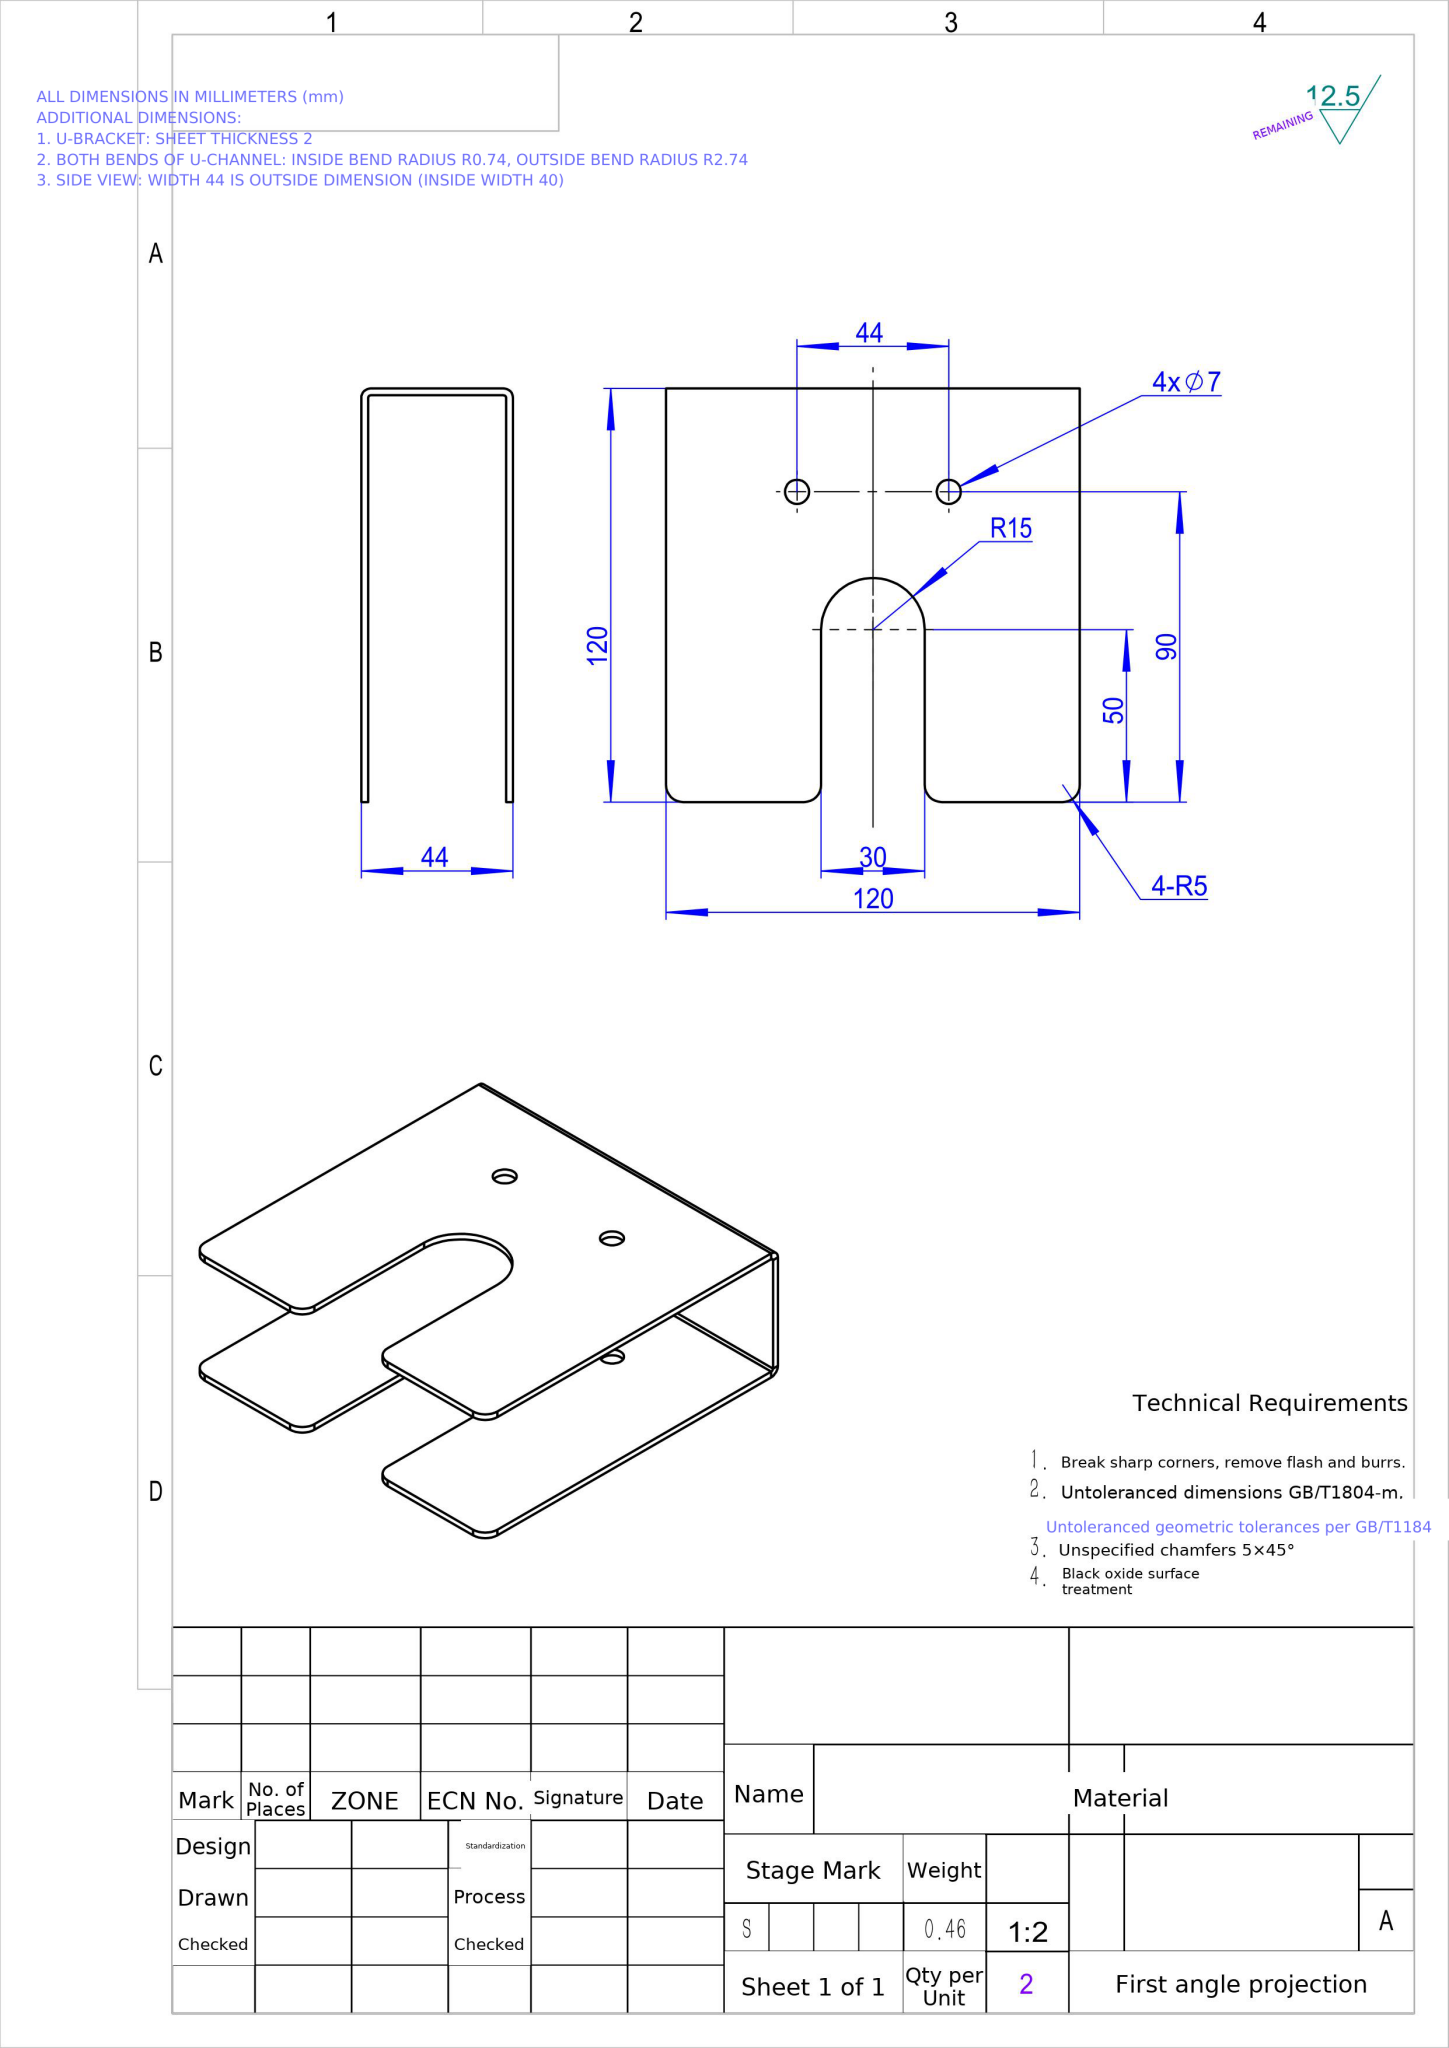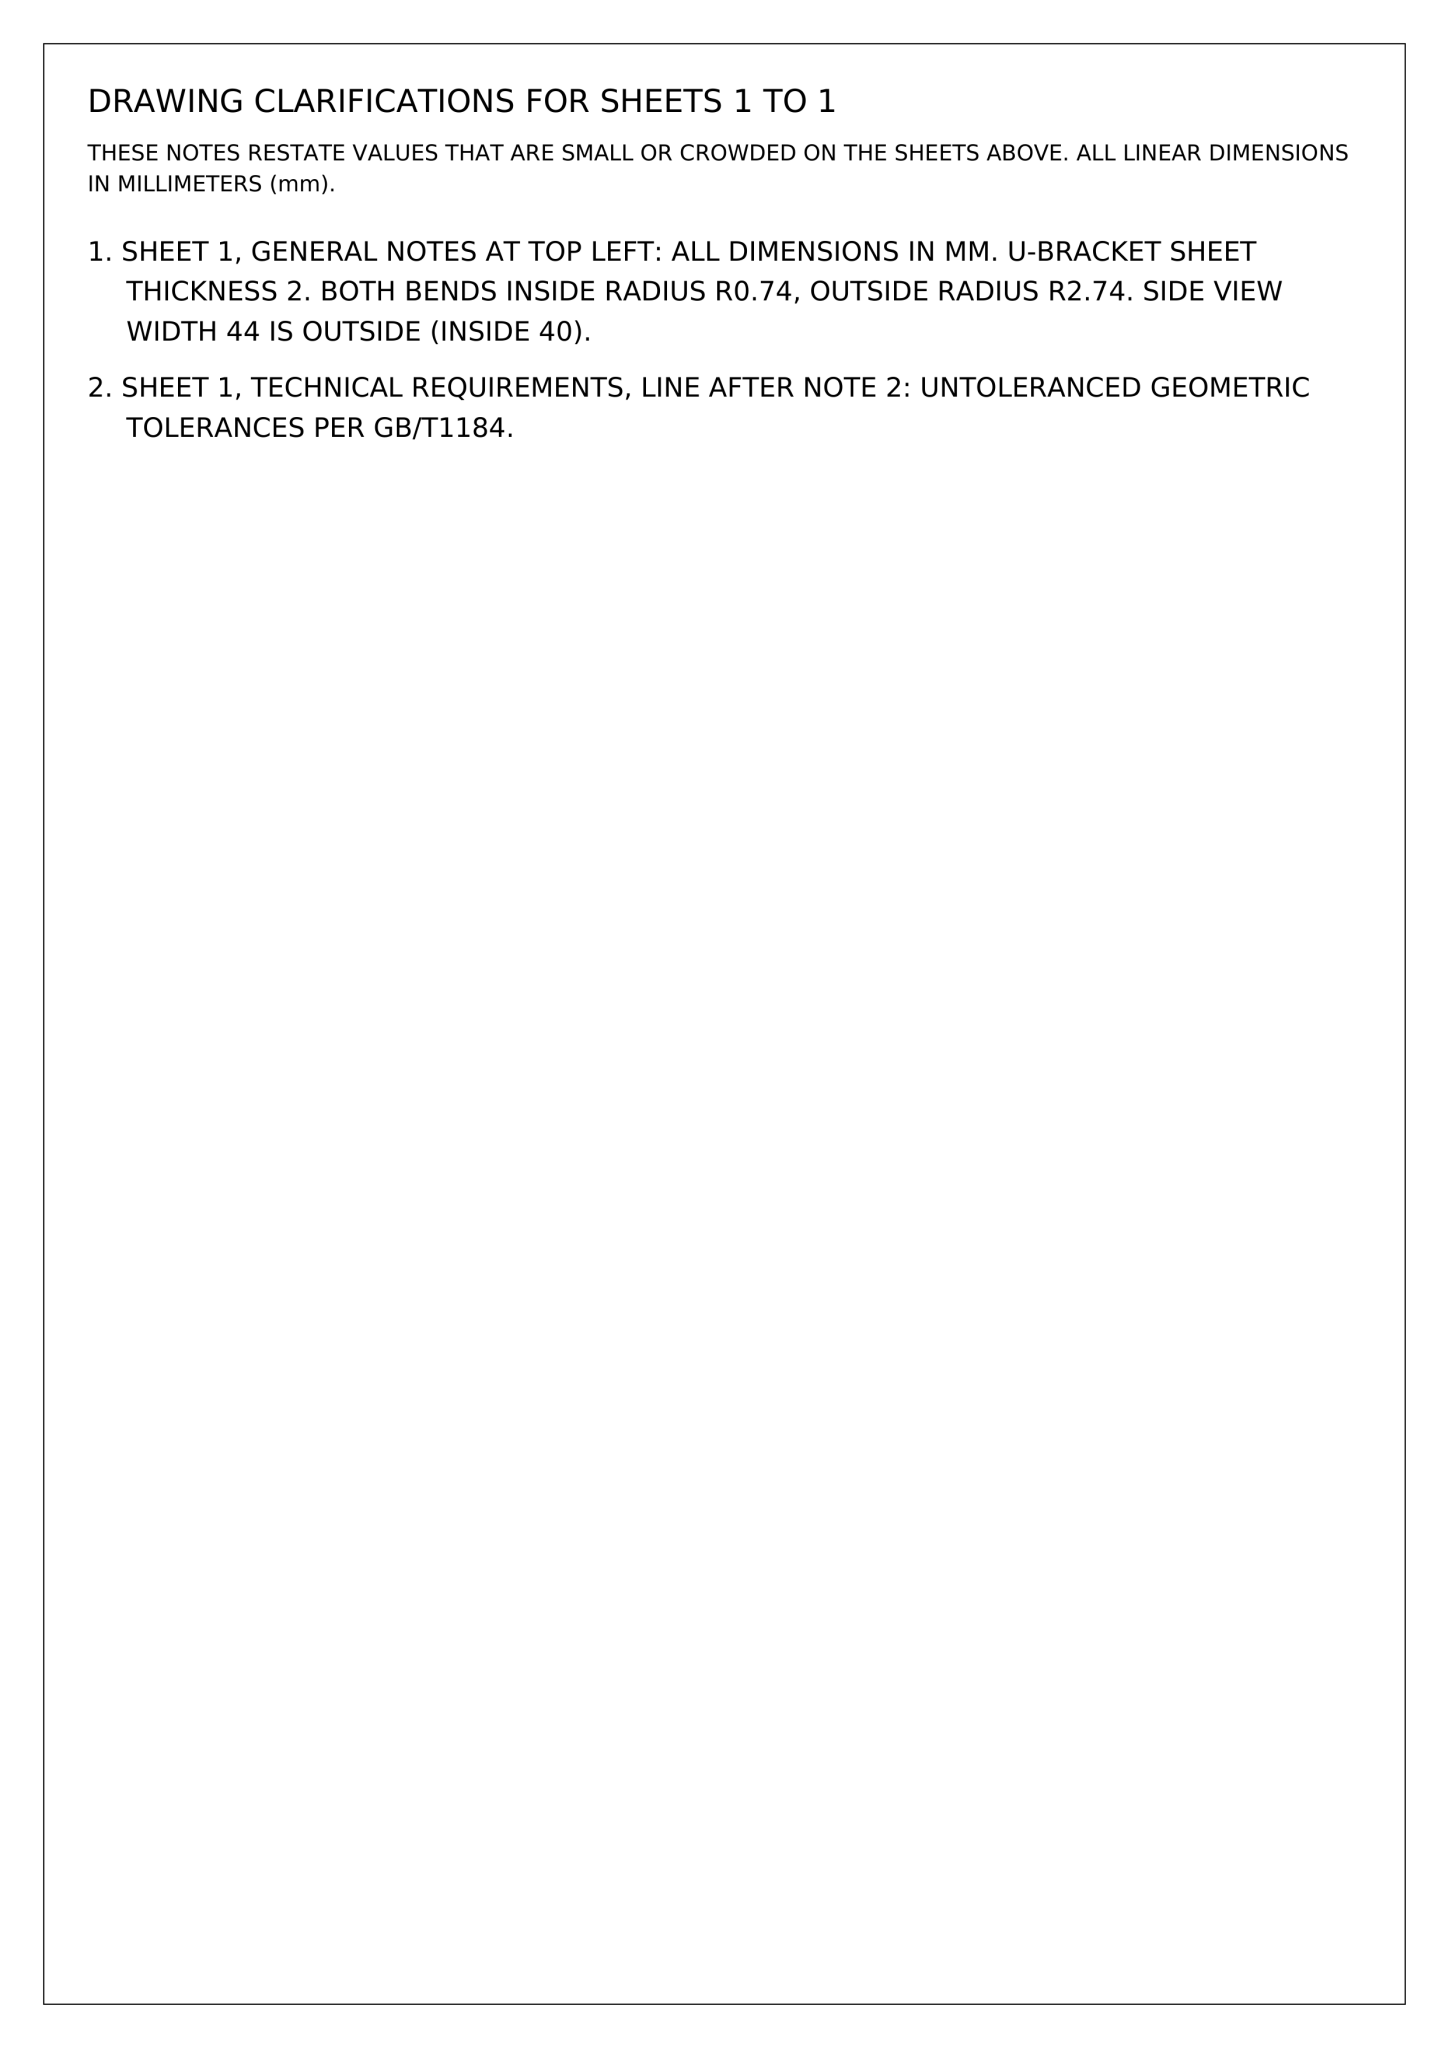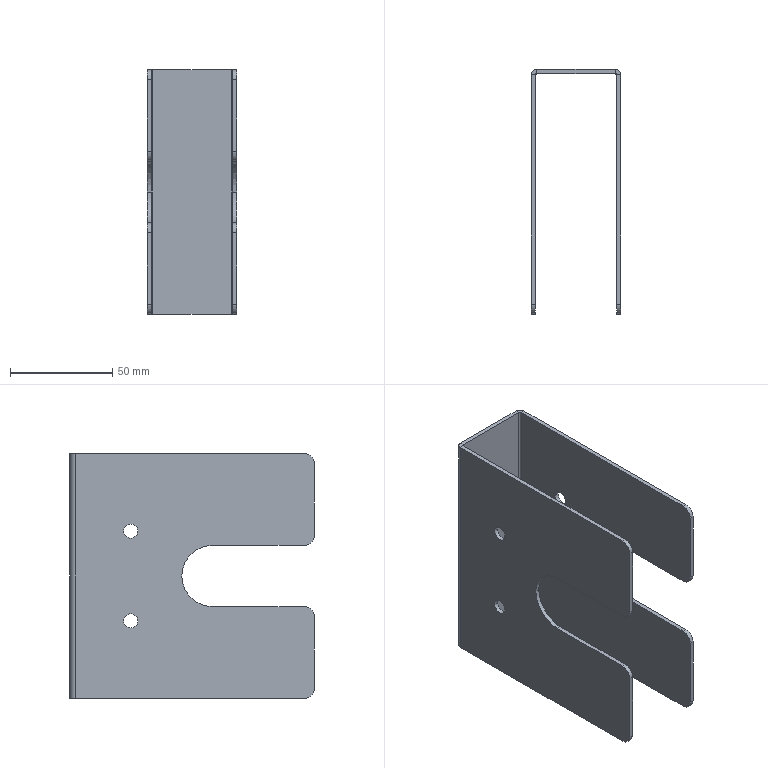Part | NX | mm | 1 solid | 48 faces | box 44 x 120 x 120 mm | volume 59035 mm3 | cylinder 24 | plane 24 | commonest cylinder face diameters 7 x8 10 x8 30 x4 5.473 x2 1.473 x2